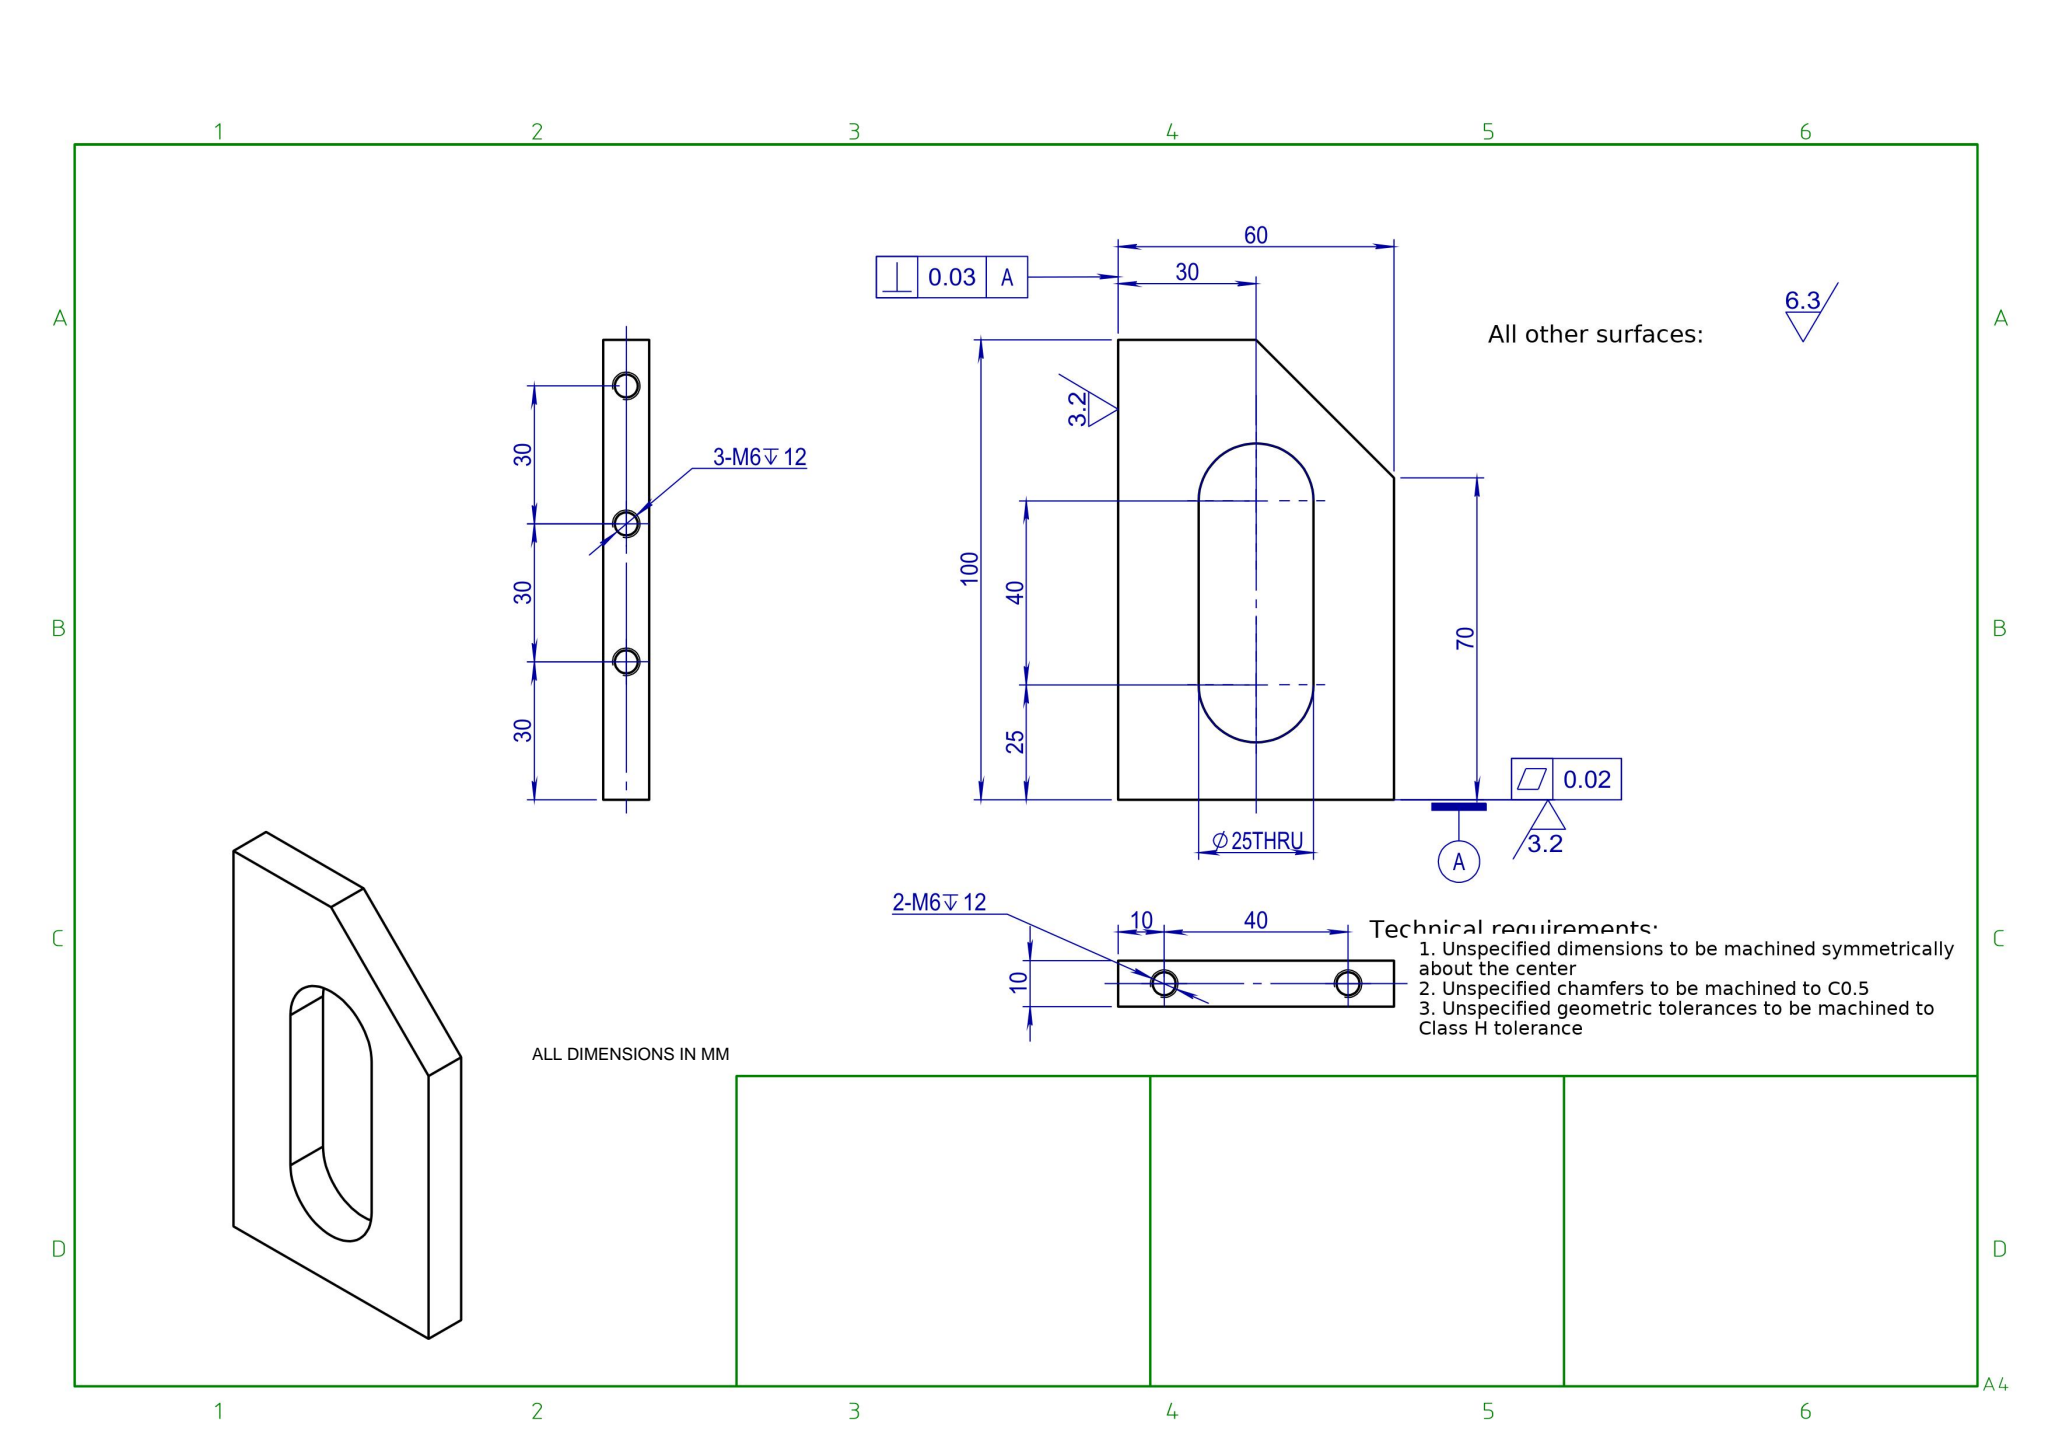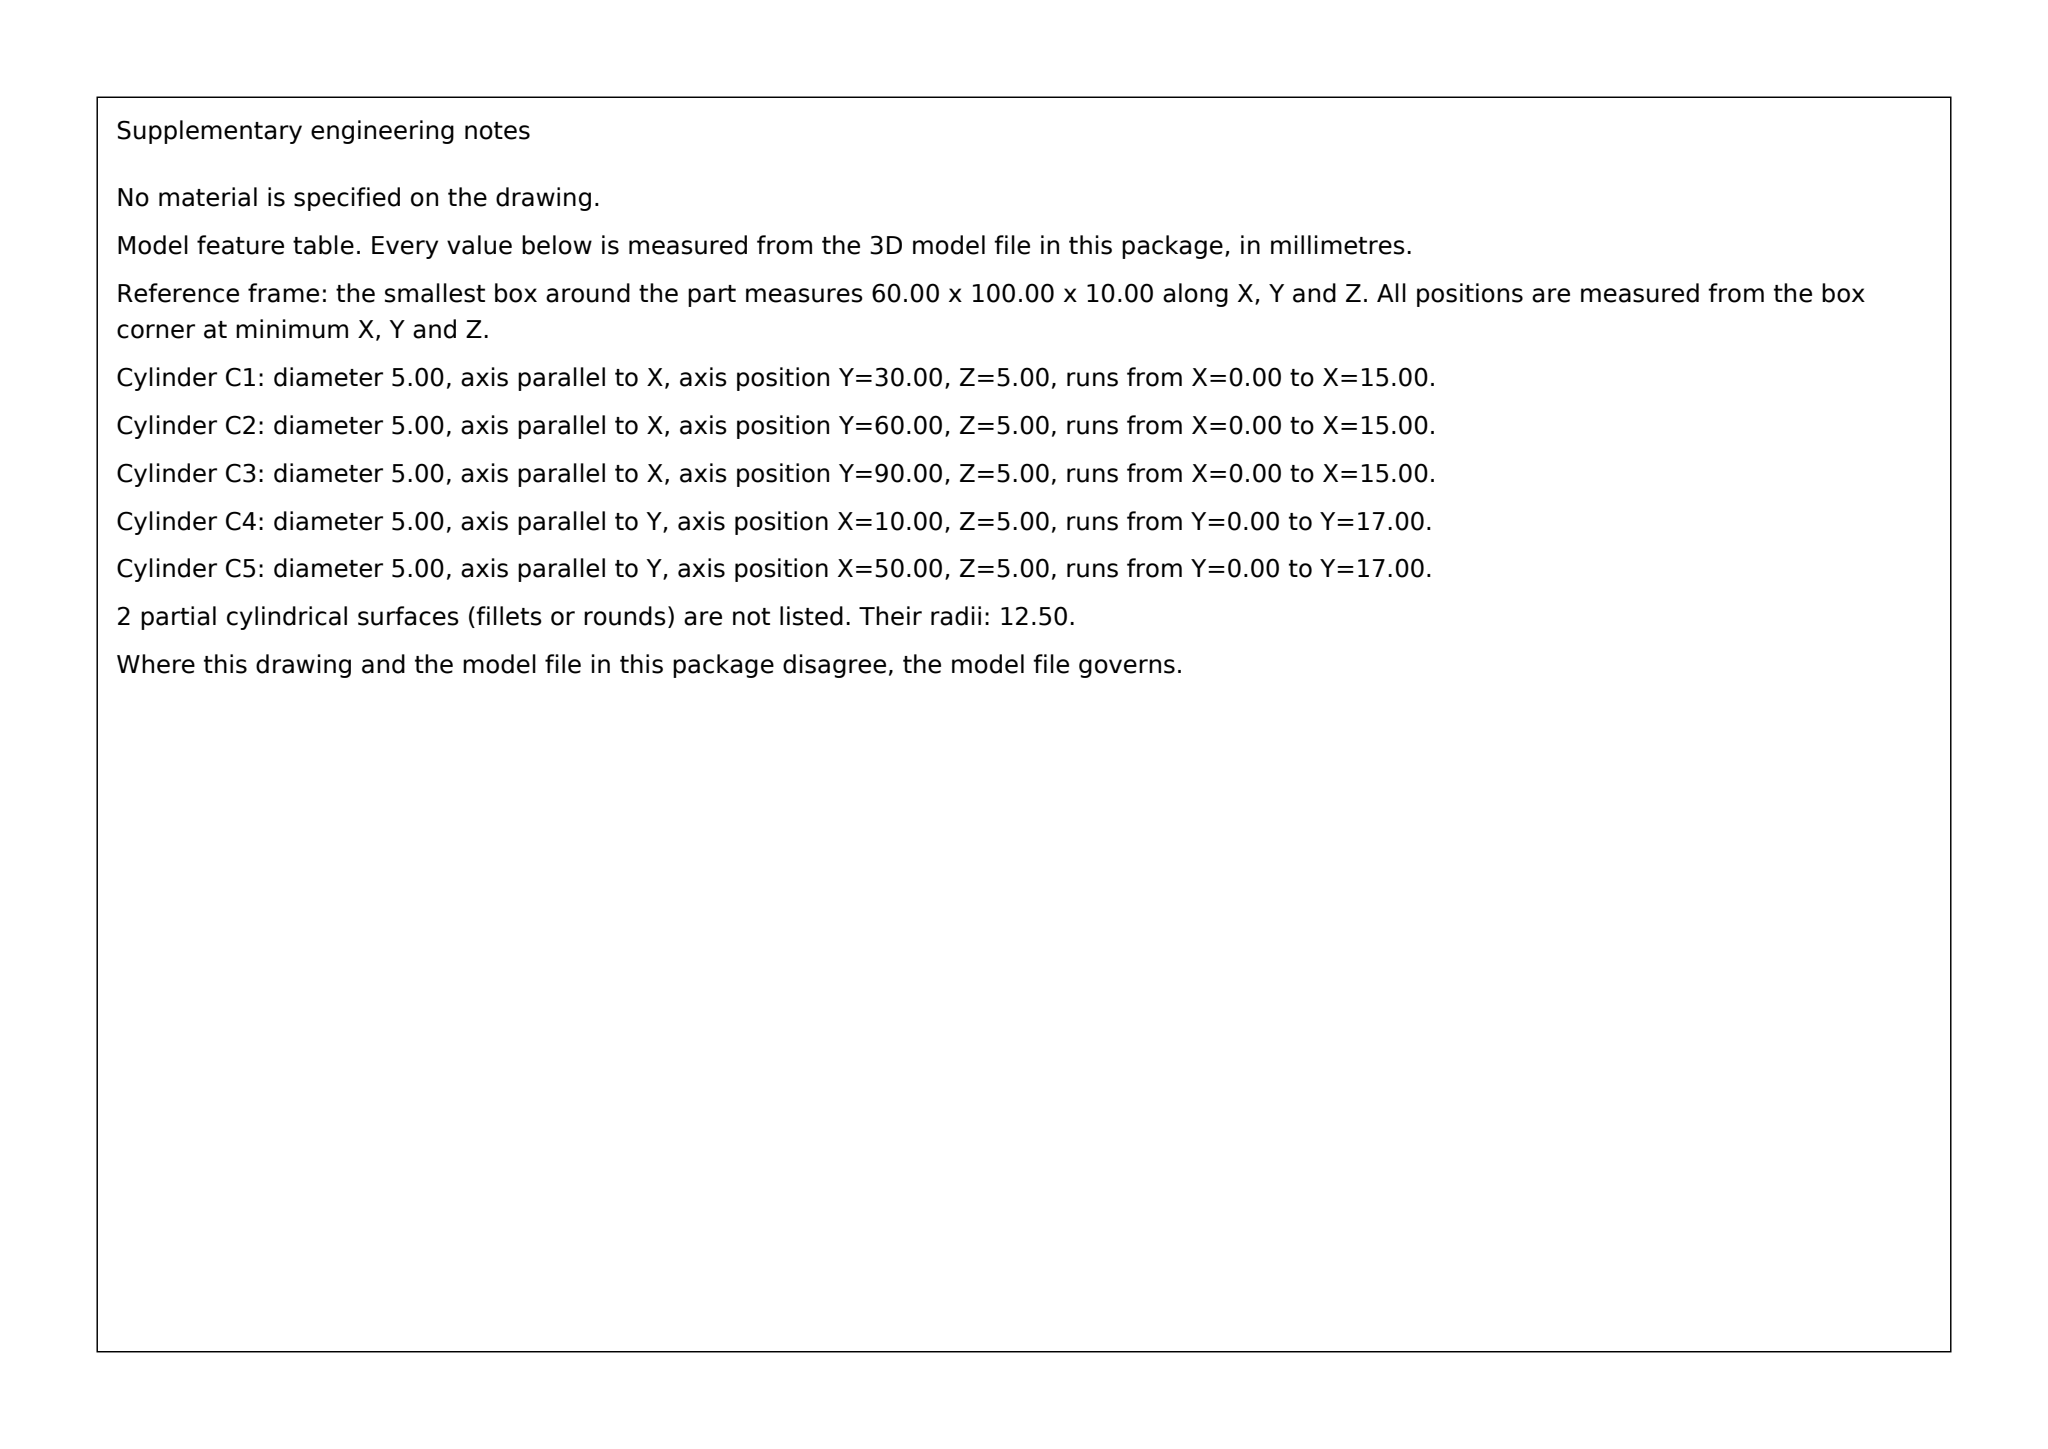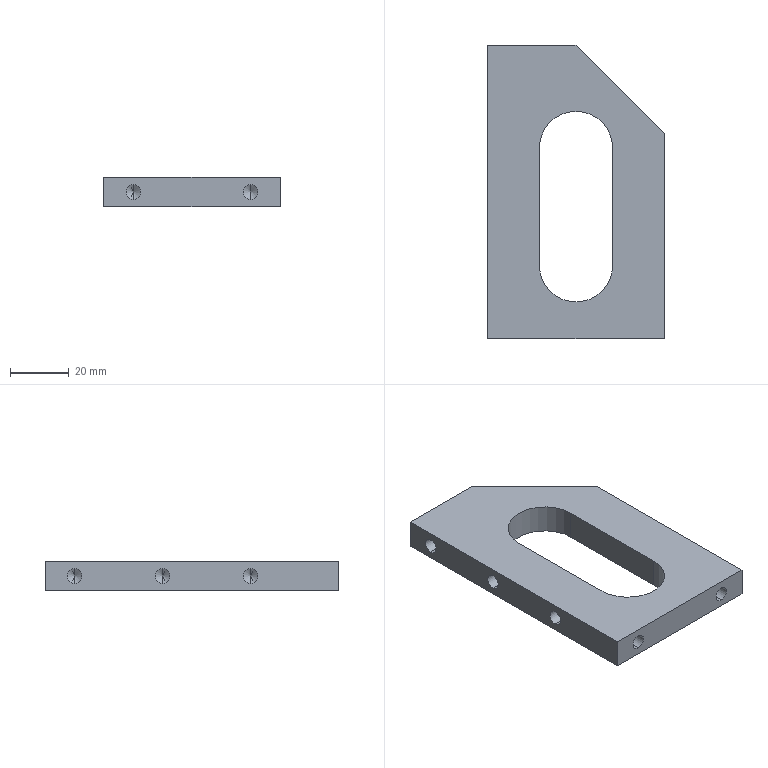Part | SolidWorks | mm | 1 solid | 31 faces | box 60 x 100 x 10 mm | volume 38991 mm3 | cylinder 12 | cone 10 | plane 9 | commonest cylinder face diameters 5 x10 25 x2
build123d program:
from build123d import *

# Parameters (mm, degrees)
EXTRUDE1_DEPTH        = 5
M6_TAPPED_HOLE1_D     = 5
M6_TAPPED_HOLE1_DEPTH = 17
M6_TAPPED_HOLE1_TIP   = 1.502
M6_TAPPED_HOLE2_D     = 5
M6_TAPPED_HOLE2_DEPTH = 15
M6_TAPPED_HOLE2_TIP   = 1.502
CUT_EXTRUDE1_DEPTH    = 118.047


with BuildPart() as part:
    # Sketch1 → Extrude1 (new, symmetric)
    with BuildSketch(Plane.XY):
        Polygon((0, 0), (60, 0), (60, 70), (30, 100), (0, 100), align=None)
    extrude(amount=EXTRUDE1_DEPTH, both=True)

    # M6 Tapped Hole1
    with Locations(Plane.XZ):
        with Locations((50, 0), (10, 0)):
            Hole(M6_TAPPED_HOLE1_D / 2, depth=M6_TAPPED_HOLE1_DEPTH)
            with Locations((0, 0, -(M6_TAPPED_HOLE1_DEPTH + M6_TAPPED_HOLE1_TIP / 2))):  # 118° drill point
                Cone(0, M6_TAPPED_HOLE1_D / 2, M6_TAPPED_HOLE1_TIP, mode=Mode.SUBTRACT)

    # M6 Tapped Hole2
    with Locations(Plane.ZY):
        with Locations((0, 30), (0, 60), (0, 90)):
            Hole(M6_TAPPED_HOLE2_D / 2, depth=M6_TAPPED_HOLE2_DEPTH)
            with Locations((0, 0, -(M6_TAPPED_HOLE2_DEPTH + M6_TAPPED_HOLE2_TIP / 2))):  # 118° drill point
                Cone(0, M6_TAPPED_HOLE2_D / 2, M6_TAPPED_HOLE2_TIP, mode=Mode.SUBTRACT)

    # Sketch8 → Cut-Extrude1 (cut, through all)
    with BuildSketch(Plane.XY.offset(5)):
        with BuildLine():
            Line((17.5, 65), (17.5, 25))
            ThreePointArc((17.5, 25), (30, 12.5), (42.5, 25))
            Line((42.5, 25), (42.5, 65))
            ThreePointArc((42.5, 65), (30, 77.5), (17.5, 65))
        make_face()
    extrude(amount=-CUT_EXTRUDE1_DEPTH, mode=Mode.SUBTRACT)


solid = part.part
STEP:
#1=CARTESIAN_POINT('',(15.,30.,-2.5));
#2=VERTEX_POINT('',#1);
#3=CARTESIAN_POINT('',(15.,30.,2.5));
#4=VERTEX_POINT('',#3);
#5=CARTESIAN_POINT('',(15.,30.,0.));
#6=DIRECTION('',(-1.,0.,0.));
#7=DIRECTION('',(0.,0.,1.));
#8=AXIS2_PLACEMENT_3D('',#5,#6,#7);
#9=CIRCLE('',#8,2.5);
#10=EDGE_CURVE('',#2,#4,#9,.T.);
#11=ORIENTED_EDGE('',*,*,#10,.F.);
#12=CARTESIAN_POINT('',(-0.,30.,-2.5));
#13=VERTEX_POINT('',#12);
#14=CARTESIAN_POINT('',(-0.,30.,-2.5));
#15=DIRECTION('',(-1.,0.,0.));
#16=VECTOR('',#15,1000.);
#17=LINE('',#14,#16);
#18=EDGE_CURVE('',#2,#13,#17,.T.);
#19=ORIENTED_EDGE('',*,*,#18,.T.);
#20=CARTESIAN_POINT('',(-0.,30.,2.5));
#21=VERTEX_POINT('',#20);
#22=CARTESIAN_POINT('',(-0.,30.,0.));
#23=DIRECTION('',(-1.,0.,0.));
#24=DIRECTION('',(0.,0.,1.));
#25=AXIS2_PLACEMENT_3D('',#22,#23,#24);
#26=CIRCLE('',#25,2.5);
#27=EDGE_CURVE('',#13,#21,#26,.T.);
#28=ORIENTED_EDGE('',*,*,#27,.T.);
#29=CARTESIAN_POINT('',(-0.,30.,2.5));
#30=DIRECTION('',(-1.,0.,0.));
#31=VECTOR('',#30,1000.);
#32=LINE('',#29,#31);
#33=EDGE_CURVE('',#4,#21,#32,.T.);
#34=ORIENTED_EDGE('',*,*,#33,.F.);
#35=EDGE_LOOP('',(#11,#19,#28,#34));
#36=FACE_OUTER_BOUND('',#35,.T.);
#37=CARTESIAN_POINT('',(-0.,30.,0.));
#38=DIRECTION('',(-1.,0.,0.));
#39=DIRECTION('',(0.,0.,1.));
#40=AXIS2_PLACEMENT_3D('',#37,#38,#39);
#41=CYLINDRICAL_SURFACE('',#40,2.5);
#42=ADVANCED_FACE('',(#36),#41,.F.);
#43=CARTESIAN_POINT('',(16.502,30.,0.));
#44=VERTEX_POINT('',#43);
#45=CARTESIAN_POINT('',(15.,30.,2.5));
#46=DIRECTION('',(-0.515,0.,0.8572));
#47=VECTOR('',#46,1000.);
#48=LINE('',#45,#47);
#49=EDGE_CURVE('',#44,#4,#48,.T.);
#50=ORIENTED_EDGE('',*,*,#49,.F.);
#51=CARTESIAN_POINT('',(15.,30.,-2.5));
#52=DIRECTION('',(-0.515,0.,-0.8572));
#53=VECTOR('',#52,1000.);
#54=LINE('',#51,#53);
#55=EDGE_CURVE('',#44,#2,#54,.T.);
#56=ORIENTED_EDGE('',*,*,#55,.T.);
#57=ORIENTED_EDGE('',*,*,#10,.T.);
#58=EDGE_LOOP('',(#50,#56,#57));
#59=FACE_OUTER_BOUND('',#58,.T.);
#60=CARTESIAN_POINT('',(15.,30.,0.));
#61=DIRECTION('',(-1.,0.,0.));
#62=DIRECTION('',(0.,0.,1.));
#63=AXIS2_PLACEMENT_3D('',#60,#61,#62);
#64=CONICAL_SURFACE('',#63,2.5,1.03);
#65=ADVANCED_FACE('',(#59),#64,.F.);
#66=CARTESIAN_POINT('',(15.,60.,-2.5));
#67=VERTEX_POINT('',#66);
#68=CARTESIAN_POINT('',(15.,60.,2.5));
#69=VERTEX_POINT('',#68);
#70=CARTESIAN_POINT('',(15.,60.,0.));
#71=DIRECTION('',(-1.,0.,0.));
#72=DIRECTION('',(0.,0.,1.));
#73=AXIS2_PLACEMENT_3D('',#70,#71,#72);
#74=CIRCLE('',#73,2.5);
#75=EDGE_CURVE('',#67,#69,#74,.T.);
#76=ORIENTED_EDGE('',*,*,#75,.F.);
#77=CARTESIAN_POINT('',(-0.,60.,-2.5));
#78=VERTEX_POINT('',#77);
#79=CARTESIAN_POINT('',(-0.,60.,-2.5));
#80=DIRECTION('',(-1.,0.,0.));
#81=VECTOR('',#80,1000.);
#82=LINE('',#79,#81);
#83=EDGE_CURVE('',#67,#78,#82,.T.);
#84=ORIENTED_EDGE('',*,*,#83,.T.);
#85=CARTESIAN_POINT('',(-0.,60.,2.5));
#86=VERTEX_POINT('',#85);
#87=CARTESIAN_POINT('',(-0.,60.,0.));
#88=DIRECTION('',(-1.,0.,0.));
#89=DIRECTION('',(0.,0.,1.));
#90=AXIS2_PLACEMENT_3D('',#87,#88,#89);
#91=CIRCLE('',#90,2.5);
#92=EDGE_CURVE('',#78,#86,#91,.T.);
#93=ORIENTED_EDGE('',*,*,#92,.T.);
#94=CARTESIAN_POINT('',(-0.,60.,2.5));
#95=DIRECTION('',(-1.,0.,0.));
#96=VECTOR('',#95,1000.);
#97=LINE('',#94,#96);
#98=EDGE_CURVE('',#69,#86,#97,.T.);
#99=ORIENTED_EDGE('',*,*,#98,.F.);
#100=EDGE_LOOP('',(#76,#84,#93,#99));
#101=FACE_OUTER_BOUND('',#100,.T.);
#102=CARTESIAN_POINT('',(-0.,60.,0.));
#103=DIRECTION('',(-1.,0.,0.));
#104=DIRECTION('',(0.,0.,1.));
#105=AXIS2_PLACEMENT_3D('',#102,#103,#104);
#106=CYLINDRICAL_SURFACE('',#105,2.5);
#107=ADVANCED_FACE('',(#101),#106,.F.);
#108=CARTESIAN_POINT('',(16.502,60.,0.));
#109=VERTEX_POINT('',#108);
#110=CARTESIAN_POINT('',(15.,60.,2.5));
#111=DIRECTION('',(-0.515,0.,0.8572));
#112=VECTOR('',#111,1000.);
#113=LINE('',#110,#112);
#114=EDGE_CURVE('',#109,#69,#113,.T.);
#115=ORIENTED_EDGE('',*,*,#114,.F.);
#116=CARTESIAN_POINT('',(15.,60.,-2.5));
#117=DIRECTION('',(-0.515,0.,-0.8572));
#118=VECTOR('',#117,1000.);
#119=LINE('',#116,#118);
#120=EDGE_CURVE('',#109,#67,#119,.T.);
#121=ORIENTED_EDGE('',*,*,#120,.T.);
#122=ORIENTED_EDGE('',*,*,#75,.T.);
#123=EDGE_LOOP('',(#115,#121,#122));
#124=FACE_OUTER_BOUND('',#123,.T.);
#125=CARTESIAN_POINT('',(15.,60.,0.));
#126=DIRECTION('',(-1.,0.,0.));
#127=DIRECTION('',(0.,0.,1.));
#128=AXIS2_PLACEMENT_3D('',#125,#126,#127);
#129=CONICAL_SURFACE('',#128,2.5,1.03);
#130=ADVANCED_FACE('',(#124),#129,.F.);
#131=CARTESIAN_POINT('',(15.,90.,-2.5));
#132=VERTEX_POINT('',#131);
#133=CARTESIAN_POINT('',(15.,90.,2.5));
#134=VERTEX_POINT('',#133);
#135=CARTESIAN_POINT('',(15.,90.,0.));
#136=DIRECTION('',(-1.,0.,0.));
#137=DIRECTION('',(0.,0.,1.));
#138=AXIS2_PLACEMENT_3D('',#135,#136,#137);
#139=CIRCLE('',#138,2.5);
#140=EDGE_CURVE('',#132,#134,#139,.T.);
#141=ORIENTED_EDGE('',*,*,#140,.F.);
#142=CARTESIAN_POINT('',(-0.,90.,-2.5));
#143=VERTEX_POINT('',#142);
#144=CARTESIAN_POINT('',(-0.,90.,-2.5));
#145=DIRECTION('',(-1.,0.,0.));
#146=VECTOR('',#145,1000.);
#147=LINE('',#144,#146);
#148=EDGE_CURVE('',#132,#143,#147,.T.);
#149=ORIENTED_EDGE('',*,*,#148,.T.);
#150=CARTESIAN_POINT('',(-0.,90.,2.5));
#151=VERTEX_POINT('',#150);
#152=CARTESIAN_POINT('',(-0.,90.,0.));
#153=DIRECTION('',(-1.,0.,0.));
#154=DIRECTION('',(0.,0.,1.));
#155=AXIS2_PLACEMENT_3D('',#152,#153,#154);
#156=CIRCLE('',#155,2.5);
#157=EDGE_CURVE('',#143,#151,#156,.T.);
#158=ORIENTED_EDGE('',*,*,#157,.T.);
#159=CARTESIAN_POINT('',(-0.,90.,2.5));
#160=DIRECTION('',(-1.,0.,0.));
#161=VECTOR('',#160,1000.);
#162=LINE('',#159,#161);
#163=EDGE_CURVE('',#134,#151,#162,.T.);
#164=ORIENTED_EDGE('',*,*,#163,.F.);
#165=EDGE_LOOP('',(#141,#149,#158,#164));
#166=FACE_OUTER_BOUND('',#165,.T.);
#167=CARTESIAN_POINT('',(-0.,90.,0.));
#168=DIRECTION('',(-1.,0.,0.));
#169=DIRECTION('',(0.,0.,1.));
#170=AXIS2_PLACEMENT_3D('',#167,#168,#169);
#171=CYLINDRICAL_SURFACE('',#170,2.5);
#172=ADVANCED_FACE('',(#166),#171,.F.);
#173=CARTESIAN_POINT('',(16.502,90.,0.));
#174=VERTEX_POINT('',#173);
#175=CARTESIAN_POINT('',(15.,90.,2.5));
#176=DIRECTION('',(-0.515,0.,0.8572));
#177=VECTOR('',#176,1000.);
#178=LINE('',#175,#177);
#179=EDGE_CURVE('',#174,#134,#178,.T.);
#180=ORIENTED_EDGE('',*,*,#179,.F.);
#181=CARTESIAN_POINT('',(15.,90.,-2.5));
#182=DIRECTION('',(-0.515,0.,-0.8572));
#183=VECTOR('',#182,1000.);
#184=LINE('',#181,#183);
#185=EDGE_CURVE('',#174,#132,#184,.T.);
#186=ORIENTED_EDGE('',*,*,#185,.T.);
#187=ORIENTED_EDGE('',*,*,#140,.T.);
#188=EDGE_LOOP('',(#180,#186,#187));
#189=FACE_OUTER_BOUND('',#188,.T.);
#190=CARTESIAN_POINT('',(15.,90.,0.));
#191=DIRECTION('',(-1.,0.,0.));
#192=DIRECTION('',(0.,0.,1.));
#193=AXIS2_PLACEMENT_3D('',#190,#191,#192);
#194=CONICAL_SURFACE('',#193,2.5,1.03);
#195=ADVANCED_FACE('',(#189),#194,.F.);
#196=CARTESIAN_POINT('',(50.,18.502,0.));
#197=VERTEX_POINT('',#196);
#198=CARTESIAN_POINT('',(50.,17.,-2.5));
#199=VERTEX_POINT('',#198);
#200=CARTESIAN_POINT('',(50.,17.,-2.5));
#201=DIRECTION('',(0.,-0.515,-0.8572));
#202=VECTOR('',#201,1000.);
#203=LINE('',#200,#202);
#204=EDGE_CURVE('',#197,#199,#203,.T.);
#205=ORIENTED_EDGE('',*,*,#204,.F.);
#206=CARTESIAN_POINT('',(50.,17.,2.5));
#207=VERTEX_POINT('',#206);
#208=CARTESIAN_POINT('',(50.,17.,2.5));
#209=DIRECTION('',(0.,-0.515,0.8572));
#210=VECTOR('',#209,1000.);
#211=LINE('',#208,#210);
#212=EDGE_CURVE('',#197,#207,#211,.T.);
#213=ORIENTED_EDGE('',*,*,#212,.T.);
#214=CARTESIAN_POINT('',(50.,17.,0.));
#215=DIRECTION('',(0.,-1.,0.));
#216=DIRECTION('',(0.,0.,-1.));
#217=AXIS2_PLACEMENT_3D('',#214,#215,#216);
#218=CIRCLE('',#217,2.5);
#219=EDGE_CURVE('',#207,#199,#218,.T.);
#220=ORIENTED_EDGE('',*,*,#219,.T.);
#221=EDGE_LOOP('',(#205,#213,#220));
#222=FACE_OUTER_BOUND('',#221,.T.);
#223=CARTESIAN_POINT('',(50.,17.,0.));
#224=DIRECTION('',(0.,-1.,0.));
#225=DIRECTION('',(0.,0.,-1.));
#226=AXIS2_PLACEMENT_3D('',#223,#224,#225);
#227=CONICAL_SURFACE('',#226,2.5,1.03);
#228=ADVANCED_FACE('',(#222),#227,.F.);
#229=ORIENTED_EDGE('',*,*,#219,.F.);
#230=CARTESIAN_POINT('',(50.,-0.,2.5));
#231=VERTEX_POINT('',#230);
#232=CARTESIAN_POINT('',(50.,0.,2.5));
#233=DIRECTION('',(0.,-1.,0.));
#234=VECTOR('',#233,1000.);
#235=LINE('',#232,#234);
#236=EDGE_CURVE('',#207,#231,#235,.T.);
#237=ORIENTED_EDGE('',*,*,#236,.T.);
#238=CARTESIAN_POINT('',(50.,-0.,-2.5));
#239=VERTEX_POINT('',#238);
#240=CARTESIAN_POINT('',(50.,-0.,0.));
#241=DIRECTION('',(0.,-1.,0.));
#242=DIRECTION('',(0.,0.,-1.));
#243=AXIS2_PLACEMENT_3D('',#240,#241,#242);
#244=CIRCLE('',#243,2.5);
#245=EDGE_CURVE('',#231,#239,#244,.T.);
#246=ORIENTED_EDGE('',*,*,#245,.T.);
#247=CARTESIAN_POINT('',(50.,0.,-2.5));
#248=DIRECTION('',(0.,-1.,0.));
#249=VECTOR('',#248,1000.);
#250=LINE('',#247,#249);
#251=EDGE_CURVE('',#199,#239,#250,.T.);
#252=ORIENTED_EDGE('',*,*,#251,.F.);
#253=EDGE_LOOP('',(#229,#237,#246,#252));
#254=FACE_OUTER_BOUND('',#253,.T.);
#255=CARTESIAN_POINT('',(50.,0.,0.));
#256=DIRECTION('',(0.,-1.,0.));
#257=DIRECTION('',(0.,0.,-1.));
#258=AXIS2_PLACEMENT_3D('',#255,#256,#257);
#259=CYLINDRICAL_SURFACE('',#258,2.5);
#260=ADVANCED_FACE('',(#254),#259,.F.);
#261=CARTESIAN_POINT('',(10.,18.502,0.));
#262=VERTEX_POINT('',#261);
#263=CARTESIAN_POINT('',(10.,17.,-2.5));
#264=VERTEX_POINT('',#263);
#265=CARTESIAN_POINT('',(10.,17.,-2.5));
#266=DIRECTION('',(0.,-0.515,-0.8572));
#267=VECTOR('',#266,1000.);
#268=LINE('',#265,#267);
#269=EDGE_CURVE('',#262,#264,#268,.T.);
#270=ORIENTED_EDGE('',*,*,#269,.F.);
#271=CARTESIAN_POINT('',(10.,17.,2.5));
#272=VERTEX_POINT('',#271);
#273=CARTESIAN_POINT('',(10.,17.,2.5));
#274=DIRECTION('',(0.,-0.515,0.8572));
#275=VECTOR('',#274,1000.);
#276=LINE('',#273,#275);
#277=EDGE_CURVE('',#262,#272,#276,.T.);
#278=ORIENTED_EDGE('',*,*,#277,.T.);
#279=CARTESIAN_POINT('',(10.,17.,0.));
#280=DIRECTION('',(0.,-1.,0.));
#281=DIRECTION('',(0.,0.,-1.));
#282=AXIS2_PLACEMENT_3D('',#279,#280,#281);
#283=CIRCLE('',#282,2.5);
#284=EDGE_CURVE('',#272,#264,#283,.T.);
#285=ORIENTED_EDGE('',*,*,#284,.T.);
#286=EDGE_LOOP('',(#270,#278,#285));
#287=FACE_OUTER_BOUND('',#286,.T.);
#288=CARTESIAN_POINT('',(10.,17.,0.));
#289=DIRECTION('',(0.,-1.,0.));
#290=DIRECTION('',(0.,0.,-1.));
#291=AXIS2_PLACEMENT_3D('',#288,#289,#290);
#292=CONICAL_SURFACE('',#291,2.5,1.03);
#293=ADVANCED_FACE('',(#287),#292,.F.);
#294=ORIENTED_EDGE('',*,*,#284,.F.);
#295=CARTESIAN_POINT('',(10.,-0.,2.5));
#296=VERTEX_POINT('',#295);
#297=CARTESIAN_POINT('',(10.,0.,2.5));
#298=DIRECTION('',(0.,-1.,0.));
#299=VECTOR('',#298,1000.);
#300=LINE('',#297,#299);
#301=EDGE_CURVE('',#272,#296,#300,.T.);
#302=ORIENTED_EDGE('',*,*,#301,.T.);
#303=CARTESIAN_POINT('',(10.,-0.,-2.5));
#304=VERTEX_POINT('',#303);
#305=CARTESIAN_POINT('',(10.,-0.,0.));
#306=DIRECTION('',(0.,-1.,0.));
#307=DIRECTION('',(0.,0.,-1.));
#308=AXIS2_PLACEMENT_3D('',#305,#306,#307);
#309=CIRCLE('',#308,2.5);
#310=EDGE_CURVE('',#296,#304,#309,.T.);
#311=ORIENTED_EDGE('',*,*,#310,.T.);
#312=CARTESIAN_POINT('',(10.,0.,-2.5));
#313=DIRECTION('',(0.,-1.,0.));
#314=VECTOR('',#313,1000.);
#315=LINE('',#312,#314);
#316=EDGE_CURVE('',#264,#304,#315,.T.);
#317=ORIENTED_EDGE('',*,*,#316,.F.);
#318=EDGE_LOOP('',(#294,#302,#311,#317));
#319=FACE_OUTER_BOUND('',#318,.T.);
#320=CARTESIAN_POINT('',(10.,0.,0.));
#321=DIRECTION('',(0.,-1.,0.));
#322=DIRECTION('',(0.,0.,-1.));
#323=AXIS2_PLACEMENT_3D('',#320,#321,#322);
#324=CYLINDRICAL_SURFACE('',#323,2.5);
#325=ADVANCED_FACE('',(#319),#324,.F.);
#326=CARTESIAN_POINT('',(-0.,30.,0.));
#327=DIRECTION('',(-1.,0.,0.));
#328=DIRECTION('',(0.,0.,1.));
#329=AXIS2_PLACEMENT_3D('',#326,#327,#328);
#330=CIRCLE('',#329,2.5);
#331=EDGE_CURVE('',#21,#13,#330,.T.);
#332=ORIENTED_EDGE('',*,*,#331,.F.);
#333=ORIENTED_EDGE('',*,*,#27,.F.);
#334=EDGE_LOOP('',(#332,#333));
#335=FACE_BOUND('',#334,.T.);
#336=CARTESIAN_POINT('',(-0.,60.,0.));
#337=DIRECTION('',(-1.,0.,0.));
#338=DIRECTION('',(0.,0.,1.));
#339=AXIS2_PLACEMENT_3D('',#336,#337,#338);
#340=CIRCLE('',#339,2.5);
#341=EDGE_CURVE('',#86,#78,#340,.T.);
#342=ORIENTED_EDGE('',*,*,#341,.F.);
#343=ORIENTED_EDGE('',*,*,#92,.F.);
#344=EDGE_LOOP('',(#342,#343));
#345=FACE_BOUND('',#344,.T.);
#346=CARTESIAN_POINT('',(-0.,90.,0.));
#347=DIRECTION('',(-1.,0.,0.));
#348=DIRECTION('',(0.,0.,1.));
#349=AXIS2_PLACEMENT_3D('',#346,#347,#348);
#350=CIRCLE('',#349,2.5);
#351=EDGE_CURVE('',#151,#143,#350,.T.);
#352=ORIENTED_EDGE('',*,*,#351,.F.);
#353=ORIENTED_EDGE('',*,*,#157,.F.);
#354=EDGE_LOOP('',(#352,#353));
#355=FACE_BOUND('',#354,.T.);
#356=CARTESIAN_POINT('',(-0.,100.,-5.));
#357=VERTEX_POINT('',#356);
#358=CARTESIAN_POINT('',(0.,0.,-5.));
#359=VERTEX_POINT('',#358);
#360=CARTESIAN_POINT('',(-0.,100.,-5.));
#361=DIRECTION('',(0.,-1.,0.));
#362=VECTOR('',#361,1000.);
#363=LINE('',#360,#362);
#364=EDGE_CURVE('',#357,#359,#363,.T.);
#365=ORIENTED_EDGE('',*,*,#364,.T.);
#366=CARTESIAN_POINT('',(0.,0.,5.));
#367=VERTEX_POINT('',#366);
#368=CARTESIAN_POINT('',(0.,0.,5.));
#369=DIRECTION('',(0.,0.,-1.));
#370=VECTOR('',#369,1000.);
#371=LINE('',#368,#370);
#372=EDGE_CURVE('',#367,#359,#371,.T.);
#373=ORIENTED_EDGE('',*,*,#372,.F.);
#374=CARTESIAN_POINT('',(-0.,100.,5.));
#375=VERTEX_POINT('',#374);
#376=CARTESIAN_POINT('',(-0.,100.,5.));
#377=DIRECTION('',(0.,-1.,0.));
#378=VECTOR('',#377,1000.);
#379=LINE('',#376,#378);
#380=EDGE_CURVE('',#375,#367,#379,.T.);
#381=ORIENTED_EDGE('',*,*,#380,.F.);
#382=CARTESIAN_POINT('',(-0.,100.,5.));
#383=DIRECTION('',(0.,0.,-1.));
#384=VECTOR('',#383,1000.);
#385=LINE('',#382,#384);
#386=EDGE_CURVE('',#375,#357,#385,.T.);
#387=ORIENTED_EDGE('',*,*,#386,.T.);
#388=EDGE_LOOP('',(#365,#373,#381,#387));
#389=FACE_OUTER_BOUND('',#388,.T.);
#390=CARTESIAN_POINT('',(-0.,100.,5.));
#391=DIRECTION('',(1.,0.,0.));
#392=DIRECTION('',(-0.,1.,0.));
#393=AXIS2_PLACEMENT_3D('',#390,#391,#392);
#394=PLANE('',#393);
#395=ADVANCED_FACE('',(#335,#345,#355,#389),#394,.F.);
#396=CARTESIAN_POINT('',(50.,-0.,0.));
#397=DIRECTION('',(0.,-1.,0.));
#398=DIRECTION('',(0.,0.,-1.));
#399=AXIS2_PLACEMENT_3D('',#396,#397,#398);
#400=CIRCLE('',#399,2.5);
#401=EDGE_CURVE('',#239,#231,#400,.T.);
#402=ORIENTED_EDGE('',*,*,#401,.F.);
#403=ORIENTED_EDGE('',*,*,#245,.F.);
#404=EDGE_LOOP('',(#402,#403));
#405=FACE_BOUND('',#404,.T.);
#406=CARTESIAN_POINT('',(10.,-0.,0.));
#407=DIRECTION('',(0.,-1.,0.));
#408=DIRECTION('',(0.,0.,-1.));
#409=AXIS2_PLACEMENT_3D('',#406,#407,#408);
#410=CIRCLE('',#409,2.5);
#411=EDGE_CURVE('',#304,#296,#410,.T.);
#412=ORIENTED_EDGE('',*,*,#411,.F.);
#413=ORIENTED_EDGE('',*,*,#310,.F.);
#414=EDGE_LOOP('',(#412,#413));
#415=FACE_BOUND('',#414,.T.);
#416=CARTESIAN_POINT('',(60.,0.,-5.));
#417=VERTEX_POINT('',#416);
#418=CARTESIAN_POINT('',(0.,0.,-5.));
#419=DIRECTION('',(1.,0.,0.));
#420=VECTOR('',#419,1000.);
#421=LINE('',#418,#420);
#422=EDGE_CURVE('',#359,#417,#421,.T.);
#423=ORIENTED_EDGE('',*,*,#422,.T.);
#424=CARTESIAN_POINT('',(60.,0.,5.));
#425=VERTEX_POINT('',#424);
#426=CARTESIAN_POINT('',(60.,0.,5.));
#427=DIRECTION('',(0.,0.,-1.));
#428=VECTOR('',#427,1000.);
#429=LINE('',#426,#428);
#430=EDGE_CURVE('',#425,#417,#429,.T.);
#431=ORIENTED_EDGE('',*,*,#430,.F.);
#432=CARTESIAN_POINT('',(0.,0.,5.));
#433=DIRECTION('',(1.,0.,0.));
#434=VECTOR('',#433,1000.);
#435=LINE('',#432,#434);
#436=EDGE_CURVE('',#367,#425,#435,.T.);
#437=ORIENTED_EDGE('',*,*,#436,.F.);
#438=ORIENTED_EDGE('',*,*,#372,.T.);
#439=EDGE_LOOP('',(#423,#431,#437,#438));
#440=FACE_OUTER_BOUND('',#439,.T.);
#441=CARTESIAN_POINT('',(0.,0.,5.));
#442=DIRECTION('',(0.,1.,0.));
#443=DIRECTION('',(0.,0.,1.));
#444=AXIS2_PLACEMENT_3D('',#441,#442,#443);
#445=PLANE('',#444);
#446=ADVANCED_FACE('',(#405,#415,#440),#445,.F.);
#447=CARTESIAN_POINT('',(60.,70.,-5.));
#448=VERTEX_POINT('',#447);
#449=CARTESIAN_POINT('',(60.,0.,-5.));
#450=DIRECTION('',(0.,1.,0.));
#451=VECTOR('',#450,1000.);
#452=LINE('',#449,#451);
#453=EDGE_CURVE('',#417,#448,#452,.T.);
#454=ORIENTED_EDGE('',*,*,#453,.T.);
#455=CARTESIAN_POINT('',(60.,70.,5.));
#456=VERTEX_POINT('',#455);
#457=CARTESIAN_POINT('',(60.,70.,5.));
#458=DIRECTION('',(0.,0.,-1.));
#459=VECTOR('',#458,1000.);
#460=LINE('',#457,#459);
#461=EDGE_CURVE('',#456,#448,#460,.T.);
#462=ORIENTED_EDGE('',*,*,#461,.F.);
#463=CARTESIAN_POINT('',(60.,0.,5.));
#464=DIRECTION('',(0.,1.,0.));
#465=VECTOR('',#464,1000.);
#466=LINE('',#463,#465);
#467=EDGE_CURVE('',#425,#456,#466,.T.);
#468=ORIENTED_EDGE('',*,*,#467,.F.);
#469=ORIENTED_EDGE('',*,*,#430,.T.);
#470=EDGE_LOOP('',(#454,#462,#468,#469));
#471=FACE_OUTER_BOUND('',#470,.T.);
#472=CARTESIAN_POINT('',(60.,0.,5.));
#473=DIRECTION('',(-1.,0.,0.));
#474=DIRECTION('',(0.,0.,1.));
#475=AXIS2_PLACEMENT_3D('',#472,#473,#474);
#476=PLANE('',#475);
#477=ADVANCED_FACE('',(#471),#476,.F.);
#478=CARTESIAN_POINT('',(30.,100.,-5.));
#479=VERTEX_POINT('',#478);
#480=CARTESIAN_POINT('',(60.,70.,-5.));
#481=DIRECTION('',(-0.7071,0.7071,0.));
#482=VECTOR('',#481,1000.);
#483=LINE('',#480,#482);
#484=EDGE_CURVE('',#448,#479,#483,.T.);
#485=ORIENTED_EDGE('',*,*,#484,.T.);
#486=CARTESIAN_POINT('',(30.,100.,5.));
#487=VERTEX_POINT('',#486);
#488=CARTESIAN_POINT('',(30.,100.,5.));
#489=DIRECTION('',(0.,0.,-1.));
#490=VECTOR('',#489,1000.);
#491=LINE('',#488,#490);
#492=EDGE_CURVE('',#487,#479,#491,.T.);
#493=ORIENTED_EDGE('',*,*,#492,.F.);
#494=CARTESIAN_POINT('',(60.,70.,5.));
#495=DIRECTION('',(-0.7071,0.7071,0.));
#496=VECTOR('',#495,1000.);
#497=LINE('',#494,#496);
#498=EDGE_CURVE('',#456,#487,#497,.T.);
#499=ORIENTED_EDGE('',*,*,#498,.F.);
#500=ORIENTED_EDGE('',*,*,#461,.T.);
#501=EDGE_LOOP('',(#485,#493,#499,#500));
#502=FACE_OUTER_BOUND('',#501,.T.);
#503=CARTESIAN_POINT('',(60.,70.,5.));
#504=DIRECTION('',(-0.7071,-0.7071,0.));
#505=DIRECTION('',(0.7071,-0.7071,0.));
#506=AXIS2_PLACEMENT_3D('',#503,#504,#505);
#507=PLANE('',#506);
#508=ADVANCED_FACE('',(#502),#507,.F.);
#509=CARTESIAN_POINT('',(30.,100.,-5.));
#510=DIRECTION('',(-1.,0.,0.));
#511=VECTOR('',#510,1000.);
#512=LINE('',#509,#511);
#513=EDGE_CURVE('',#479,#357,#512,.T.);
#514=ORIENTED_EDGE('',*,*,#513,.T.);
#515=ORIENTED_EDGE('',*,*,#386,.F.);
#516=CARTESIAN_POINT('',(30.,100.,5.));
#517=DIRECTION('',(-1.,0.,0.));
#518=VECTOR('',#517,1000.);
#519=LINE('',#516,#518);
#520=EDGE_CURVE('',#487,#375,#519,.T.);
#521=ORIENTED_EDGE('',*,*,#520,.F.);
#522=ORIENTED_EDGE('',*,*,#492,.T.);
#523=EDGE_LOOP('',(#514,#515,#521,#522));
#524=FACE_OUTER_BOUND('',#523,.T.);
#525=CARTESIAN_POINT('',(30.,100.,5.));
#526=DIRECTION('',(0.,-1.,0.));
#527=DIRECTION('',(0.,0.,-1.));
#528=AXIS2_PLACEMENT_3D('',#525,#526,#527);
#529=PLANE('',#528);
#530=ADVANCED_FACE('',(#524),#529,.F.);
#531=CARTESIAN_POINT('',(17.5,65.,5.));
#532=VERTEX_POINT('',#531);
#533=CARTESIAN_POINT('',(17.5,25.,5.));
#534=VERTEX_POINT('',#533);
#535=CARTESIAN_POINT('',(17.5,65.,5.));
#536=DIRECTION('',(0.,-1.,0.));
#537=VECTOR('',#536,1000.);
#538=LINE('',#535,#537);
#539=EDGE_CURVE('',#532,#534,#538,.T.);
#540=ORIENTED_EDGE('',*,*,#539,.F.);
#541=CARTESIAN_POINT('',(42.5,65.,5.));
#542=VERTEX_POINT('',#541);
#543=CARTESIAN_POINT('',(30.,65.,5.));
#544=DIRECTION('',(0.,0.,1.));
#545=DIRECTION('',(1.,0.,0.));
#546=AXIS2_PLACEMENT_3D('',#543,#544,#545);
#547=CIRCLE('',#546,12.5);
#548=EDGE_CURVE('',#542,#532,#547,.T.);
#549=ORIENTED_EDGE('',*,*,#548,.F.);
#550=CARTESIAN_POINT('',(42.5,25.,5.));
#551=VERTEX_POINT('',#550);
#552=CARTESIAN_POINT('',(42.5,65.,5.));
#553=DIRECTION('',(-0.,1.,0.));
#554=VECTOR('',#553,1000.);
#555=LINE('',#552,#554);
#556=EDGE_CURVE('',#551,#542,#555,.T.);
#557=ORIENTED_EDGE('',*,*,#556,.F.);
#558=CARTESIAN_POINT('',(30.,25.,5.));
#559=DIRECTION('',(0.,0.,1.));
#560=DIRECTION('',(1.,0.,0.));
#561=AXIS2_PLACEMENT_3D('',#558,#559,#560);
#562=CIRCLE('',#561,12.5);
#563=EDGE_CURVE('',#534,#551,#562,.T.);
#564=ORIENTED_EDGE('',*,*,#563,.F.);
#565=EDGE_LOOP('',(#540,#549,#557,#564));
#566=FACE_BOUND('',#565,.T.);
#567=ORIENTED_EDGE('',*,*,#380,.T.);
#568=ORIENTED_EDGE('',*,*,#436,.T.);
#569=ORIENTED_EDGE('',*,*,#467,.T.);
#570=ORIENTED_EDGE('',*,*,#498,.T.);
#571=ORIENTED_EDGE('',*,*,#520,.T.);
#572=EDGE_LOOP('',(#567,#568,#569,#570,#571));
#573=FACE_OUTER_BOUND('',#572,.T.);
#574=CARTESIAN_POINT('',(0.,100.,5.));
#575=DIRECTION('',(0.,0.,-1.));
#576=DIRECTION('',(-1.,0.,0.));
#577=AXIS2_PLACEMENT_3D('',#574,#575,#576);
#578=PLANE('',#577);
#579=ADVANCED_FACE('',(#566,#573),#578,.F.);
#580=CARTESIAN_POINT('',(42.5,65.,-5.));
#581=VERTEX_POINT('',#580);
#582=CARTESIAN_POINT('',(17.5,65.,-5.));
#583=VERTEX_POINT('',#582);
#584=CARTESIAN_POINT('',(30.,65.,-5.));
#585=DIRECTION('',(0.,0.,1.));
#586=DIRECTION('',(1.,0.,0.));
#587=AXIS2_PLACEMENT_3D('',#584,#585,#586);
#588=CIRCLE('',#587,12.5);
#589=EDGE_CURVE('',#581,#583,#588,.T.);
#590=ORIENTED_EDGE('',*,*,#589,.T.);
#591=CARTESIAN_POINT('',(17.5,25.,-5.));
#592=VERTEX_POINT('',#591);
#593=CARTESIAN_POINT('',(17.5,65.,-5.));
#594=DIRECTION('',(0.,-1.,0.));
#595=VECTOR('',#594,1000.);
#596=LINE('',#593,#595);
#597=EDGE_CURVE('',#583,#592,#596,.T.);
#598=ORIENTED_EDGE('',*,*,#597,.T.);
#599=CARTESIAN_POINT('',(42.5,25.,-5.));
#600=VERTEX_POINT('',#599);
#601=CARTESIAN_POINT('',(30.,25.,-5.));
#602=DIRECTION('',(0.,0.,1.));
#603=DIRECTION('',(1.,0.,0.));
#604=AXIS2_PLACEMENT_3D('',#601,#602,#603);
#605=CIRCLE('',#604,12.5);
#606=EDGE_CURVE('',#592,#600,#605,.T.);
#607=ORIENTED_EDGE('',*,*,#606,.T.);
#608=CARTESIAN_POINT('',(42.5,65.,-5.));
#609=DIRECTION('',(-0.,1.,0.));
#610=VECTOR('',#609,1000.);
#611=LINE('',#608,#610);
#612=EDGE_CURVE('',#600,#581,#611,.T.);
#613=ORIENTED_EDGE('',*,*,#612,.T.);
#614=EDGE_LOOP('',(#590,#598,#607,#613));
#615=FACE_BOUND('',#614,.T.);
#616=ORIENTED_EDGE('',*,*,#364,.F.);
#617=ORIENTED_EDGE('',*,*,#513,.F.);
#618=ORIENTED_EDGE('',*,*,#484,.F.);
#619=ORIENTED_EDGE('',*,*,#453,.F.);
#620=ORIENTED_EDGE('',*,*,#422,.F.);
#621=EDGE_LOOP('',(#616,#617,#618,#619,#620));
#622=FACE_OUTER_BOUND('',#621,.T.);
#623=CARTESIAN_POINT('',(0.,100.,-5.));
#624=DIRECTION('',(0.,0.,-1.));
#625=DIRECTION('',(-1.,0.,0.));
#626=AXIS2_PLACEMENT_3D('',#623,#624,#625);
#627=PLANE('',#626);
#628=ADVANCED_FACE('',(#615,#622),#627,.T.);
#629=ORIENTED_EDGE('',*,*,#301,.F.);
#630=CARTESIAN_POINT('',(10.,17.,0.));
#631=DIRECTION('',(0.,-1.,0.));
#632=DIRECTION('',(0.,0.,-1.));
#633=AXIS2_PLACEMENT_3D('',#630,#631,#632);
#634=CIRCLE('',#633,2.5);
#635=EDGE_CURVE('',#264,#272,#634,.T.);
#636=ORIENTED_EDGE('',*,*,#635,.F.);
#637=ORIENTED_EDGE('',*,*,#316,.T.);
#638=ORIENTED_EDGE('',*,*,#411,.T.);
#639=EDGE_LOOP('',(#629,#636,#637,#638));
#640=FACE_OUTER_BOUND('',#639,.T.);
#641=CARTESIAN_POINT('',(10.,0.,0.));
#642=DIRECTION('',(0.,-1.,0.));
#643=DIRECTION('',(0.,0.,-1.));
#644=AXIS2_PLACEMENT_3D('',#641,#642,#643);
#645=CYLINDRICAL_SURFACE('',#644,2.5);
#646=ADVANCED_FACE('',(#640),#645,.F.);
#647=ORIENTED_EDGE('',*,*,#277,.F.);
#648=ORIENTED_EDGE('',*,*,#269,.T.);
#649=ORIENTED_EDGE('',*,*,#635,.T.);
#650=EDGE_LOOP('',(#647,#648,#649));
#651=FACE_OUTER_BOUND('',#650,.T.);
#652=CARTESIAN_POINT('',(10.,17.,0.));
#653=DIRECTION('',(0.,-1.,0.));
#654=DIRECTION('',(0.,0.,-1.));
#655=AXIS2_PLACEMENT_3D('',#652,#653,#654);
#656=CONICAL_SURFACE('',#655,2.5,1.03);
#657=ADVANCED_FACE('',(#651),#656,.F.);
#658=ORIENTED_EDGE('',*,*,#236,.F.);
#659=CARTESIAN_POINT('',(50.,17.,0.));
#660=DIRECTION('',(0.,-1.,0.));
#661=DIRECTION('',(0.,0.,-1.));
#662=AXIS2_PLACEMENT_3D('',#659,#660,#661);
#663=CIRCLE('',#662,2.5);
#664=EDGE_CURVE('',#199,#207,#663,.T.);
#665=ORIENTED_EDGE('',*,*,#664,.F.);
#666=ORIENTED_EDGE('',*,*,#251,.T.);
#667=ORIENTED_EDGE('',*,*,#401,.T.);
#668=EDGE_LOOP('',(#658,#665,#666,#667));
#669=FACE_OUTER_BOUND('',#668,.T.);
#670=CARTESIAN_POINT('',(50.,0.,0.));
#671=DIRECTION('',(0.,-1.,0.));
#672=DIRECTION('',(0.,0.,-1.));
#673=AXIS2_PLACEMENT_3D('',#670,#671,#672);
#674=CYLINDRICAL_SURFACE('',#673,2.5);
#675=ADVANCED_FACE('',(#669),#674,.F.);
#676=ORIENTED_EDGE('',*,*,#212,.F.);
#677=ORIENTED_EDGE('',*,*,#204,.T.);
#678=ORIENTED_EDGE('',*,*,#664,.T.);
#679=EDGE_LOOP('',(#676,#677,#678));
#680=FACE_OUTER_BOUND('',#679,.T.);
#681=CARTESIAN_POINT('',(50.,17.,0.));
#682=DIRECTION('',(0.,-1.,0.));
#683=DIRECTION('',(0.,0.,-1.));
#684=AXIS2_PLACEMENT_3D('',#681,#682,#683);
#685=CONICAL_SURFACE('',#684,2.5,1.03);
#686=ADVANCED_FACE('',(#680),#685,.F.);
#687=ORIENTED_EDGE('',*,*,#185,.F.);
#688=ORIENTED_EDGE('',*,*,#179,.T.);
#689=CARTESIAN_POINT('',(15.,90.,0.));
#690=DIRECTION('',(-1.,0.,0.));
#691=DIRECTION('',(0.,0.,1.));
#692=AXIS2_PLACEMENT_3D('',#689,#690,#691);
#693=CIRCLE('',#692,2.5);
#694=EDGE_CURVE('',#134,#132,#693,.T.);
#695=ORIENTED_EDGE('',*,*,#694,.T.);
#696=EDGE_LOOP('',(#687,#688,#695));
#697=FACE_OUTER_BOUND('',#696,.T.);
#698=CARTESIAN_POINT('',(15.,90.,0.));
#699=DIRECTION('',(-1.,0.,0.));
#700=DIRECTION('',(0.,0.,1.));
#701=AXIS2_PLACEMENT_3D('',#698,#699,#700);
#702=CONICAL_SURFACE('',#701,2.5,1.03);
#703=ADVANCED_FACE('',(#697),#702,.F.);
#704=ORIENTED_EDGE('',*,*,#148,.F.);
#705=ORIENTED_EDGE('',*,*,#694,.F.);
#706=ORIENTED_EDGE('',*,*,#163,.T.);
#707=ORIENTED_EDGE('',*,*,#351,.T.);
#708=EDGE_LOOP('',(#704,#705,#706,#707));
#709=FACE_OUTER_BOUND('',#708,.T.);
#710=CARTESIAN_POINT('',(-0.,90.,0.));
#711=DIRECTION('',(-1.,0.,0.));
#712=DIRECTION('',(0.,0.,1.));
#713=AXIS2_PLACEMENT_3D('',#710,#711,#712);
#714=CYLINDRICAL_SURFACE('',#713,2.5);
#715=ADVANCED_FACE('',(#709),#714,.F.);
#716=ORIENTED_EDGE('',*,*,#120,.F.);
#717=ORIENTED_EDGE('',*,*,#114,.T.);
#718=CARTESIAN_POINT('',(15.,60.,0.));
#719=DIRECTION('',(-1.,0.,0.));
#720=DIRECTION('',(0.,0.,1.));
#721=AXIS2_PLACEMENT_3D('',#718,#719,#720);
#722=CIRCLE('',#721,2.5);
#723=EDGE_CURVE('',#69,#67,#722,.T.);
#724=ORIENTED_EDGE('',*,*,#723,.T.);
#725=EDGE_LOOP('',(#716,#717,#724));
#726=FACE_OUTER_BOUND('',#725,.T.);
#727=CARTESIAN_POINT('',(15.,60.,0.));
#728=DIRECTION('',(-1.,0.,0.));
#729=DIRECTION('',(0.,0.,1.));
#730=AXIS2_PLACEMENT_3D('',#727,#728,#729);
#731=CONICAL_SURFACE('',#730,2.5,1.03);
#732=ADVANCED_FACE('',(#726),#731,.F.);
#733=ORIENTED_EDGE('',*,*,#83,.F.);
#734=ORIENTED_EDGE('',*,*,#723,.F.);
#735=ORIENTED_EDGE('',*,*,#98,.T.);
#736=ORIENTED_EDGE('',*,*,#341,.T.);
#737=EDGE_LOOP('',(#733,#734,#735,#736));
#738=FACE_OUTER_BOUND('',#737,.T.);
#739=CARTESIAN_POINT('',(-0.,60.,0.));
#740=DIRECTION('',(-1.,0.,0.));
#741=DIRECTION('',(0.,0.,1.));
#742=AXIS2_PLACEMENT_3D('',#739,#740,#741);
#743=CYLINDRICAL_SURFACE('',#742,2.5);
#744=ADVANCED_FACE('',(#738),#743,.F.);
#745=ORIENTED_EDGE('',*,*,#55,.F.);
#746=ORIENTED_EDGE('',*,*,#49,.T.);
#747=CARTESIAN_POINT('',(15.,30.,0.));
#748=DIRECTION('',(-1.,0.,0.));
#749=DIRECTION('',(0.,0.,1.));
#750=AXIS2_PLACEMENT_3D('',#747,#748,#749);
#751=CIRCLE('',#750,2.5);
#752=EDGE_CURVE('',#4,#2,#751,.T.);
#753=ORIENTED_EDGE('',*,*,#752,.T.);
#754=EDGE_LOOP('',(#745,#746,#753));
#755=FACE_OUTER_BOUND('',#754,.T.);
#756=CARTESIAN_POINT('',(15.,30.,0.));
#757=DIRECTION('',(-1.,0.,0.));
#758=DIRECTION('',(0.,0.,1.));
#759=AXIS2_PLACEMENT_3D('',#756,#757,#758);
#760=CONICAL_SURFACE('',#759,2.5,1.03);
#761=ADVANCED_FACE('',(#755),#760,.F.);
#762=ORIENTED_EDGE('',*,*,#18,.F.);
#763=ORIENTED_EDGE('',*,*,#752,.F.);
#764=ORIENTED_EDGE('',*,*,#33,.T.);
#765=ORIENTED_EDGE('',*,*,#331,.T.);
#766=EDGE_LOOP('',(#762,#763,#764,#765));
#767=FACE_OUTER_BOUND('',#766,.T.);
#768=CARTESIAN_POINT('',(-0.,30.,0.));
#769=DIRECTION('',(-1.,0.,0.));
#770=DIRECTION('',(0.,0.,1.));
#771=AXIS2_PLACEMENT_3D('',#768,#769,#770);
#772=CYLINDRICAL_SURFACE('',#771,2.5);
#773=ADVANCED_FACE('',(#767),#772,.F.);
#774=ORIENTED_EDGE('',*,*,#548,.T.);
#775=CARTESIAN_POINT('',(17.5,65.,-5.));
#776=DIRECTION('',(0.,0.,1.));
#777=VECTOR('',#776,1000.);
#778=LINE('',#775,#777);
#779=EDGE_CURVE('',#583,#532,#778,.T.);
#780=ORIENTED_EDGE('',*,*,#779,.F.);
#781=ORIENTED_EDGE('',*,*,#589,.F.);
#782=CARTESIAN_POINT('',(42.5,65.,-5.));
#783=DIRECTION('',(0.,0.,1.));
#784=VECTOR('',#783,1000.);
#785=LINE('',#782,#784);
#786=EDGE_CURVE('',#581,#542,#785,.T.);
#787=ORIENTED_EDGE('',*,*,#786,.T.);
#788=EDGE_LOOP('',(#774,#780,#781,#787));
#789=FACE_OUTER_BOUND('',#788,.T.);
#790=CARTESIAN_POINT('',(30.,65.,-5.));
#791=DIRECTION('',(0.,0.,1.));
#792=DIRECTION('',(1.,0.,0.));
#793=AXIS2_PLACEMENT_3D('',#790,#791,#792);
#794=CYLINDRICAL_SURFACE('',#793,12.5);
#795=ADVANCED_FACE('',(#789),#794,.F.);
#796=ORIENTED_EDGE('',*,*,#556,.T.);
#797=ORIENTED_EDGE('',*,*,#786,.F.);
#798=ORIENTED_EDGE('',*,*,#612,.F.);
#799=CARTESIAN_POINT('',(42.5,25.,-5.));
#800=DIRECTION('',(0.,0.,1.));
#801=VECTOR('',#800,1000.);
#802=LINE('',#799,#801);
#803=EDGE_CURVE('',#600,#551,#802,.T.);
#804=ORIENTED_EDGE('',*,*,#803,.T.);
#805=EDGE_LOOP('',(#796,#797,#798,#804));
#806=FACE_OUTER_BOUND('',#805,.T.);
#807=CARTESIAN_POINT('',(42.5,65.,-5.));
#808=DIRECTION('',(1.,0.,0.));
#809=DIRECTION('',(-0.,1.,0.));
#810=AXIS2_PLACEMENT_3D('',#807,#808,#809);
#811=PLANE('',#810);
#812=ADVANCED_FACE('',(#806),#811,.F.);
#813=ORIENTED_EDGE('',*,*,#563,.T.);
#814=ORIENTED_EDGE('',*,*,#803,.F.);
#815=ORIENTED_EDGE('',*,*,#606,.F.);
#816=CARTESIAN_POINT('',(17.5,25.,-5.));
#817=DIRECTION('',(0.,0.,1.));
#818=VECTOR('',#817,1000.);
#819=LINE('',#816,#818);
#820=EDGE_CURVE('',#592,#534,#819,.T.);
#821=ORIENTED_EDGE('',*,*,#820,.T.);
#822=EDGE_LOOP('',(#813,#814,#815,#821));
#823=FACE_OUTER_BOUND('',#822,.T.);
#824=CARTESIAN_POINT('',(30.,25.,-5.));
#825=DIRECTION('',(0.,0.,1.));
#826=DIRECTION('',(1.,0.,0.));
#827=AXIS2_PLACEMENT_3D('',#824,#825,#826);
#828=CYLINDRICAL_SURFACE('',#827,12.5);
#829=ADVANCED_FACE('',(#823),#828,.F.);
#830=ORIENTED_EDGE('',*,*,#539,.T.);
#831=ORIENTED_EDGE('',*,*,#820,.F.);
#832=ORIENTED_EDGE('',*,*,#597,.F.);
#833=ORIENTED_EDGE('',*,*,#779,.T.);
#834=EDGE_LOOP('',(#830,#831,#832,#833));
#835=FACE_OUTER_BOUND('',#834,.T.);
#836=CARTESIAN_POINT('',(17.5,65.,-5.));
#837=DIRECTION('',(-1.,-0.,0.));
#838=DIRECTION('',(0.,-1.,0.));
#839=AXIS2_PLACEMENT_3D('',#836,#837,#838);
#840=PLANE('',#839);
#841=ADVANCED_FACE('',(#835),#840,.F.);
#842=CLOSED_SHELL('',(#42,#65,#107,#130,#172,#195,#228,#260,#293,#325,#395,#446,#477,#508,#530,#579,#628,#646,#657,#675,#686,#703,#715,#732,#744,#761,#773,#795,#812,#829,#841));
#843=MANIFOLD_SOLID_BREP('',#842);
#844=CARTESIAN_POINT('',(0.,0.,0.));
#845=DIRECTION('',(0.,0.,1.));
#846=DIRECTION('',(1.,0.,0.));
#847=AXIS2_PLACEMENT_3D('',#844,#845,#846);
#848=(LENGTH_UNIT()NAMED_UNIT(*)SI_UNIT(.MILLI.,.METRE.));
#849=UNCERTAINTY_MEASURE_WITH_UNIT(LENGTH_MEASURE(0.00001),#848,'','');
#850=(NAMED_UNIT(*)PLANE_ANGLE_UNIT()SI_UNIT($,.RADIAN.));
#851=(NAMED_UNIT(*)SI_UNIT($,.STERADIAN.)SOLID_ANGLE_UNIT());
#852=(GEOMETRIC_REPRESENTATION_CONTEXT(3)GLOBAL_UNCERTAINTY_ASSIGNED_CONTEXT((#849))GLOBAL_UNIT_ASSIGNED_CONTEXT((#848,#850,#851))REPRESENTATION_CONTEXT('',''));
#853=ADVANCED_BREP_SHAPE_REPRESENTATION('',(#843,#847),#852);